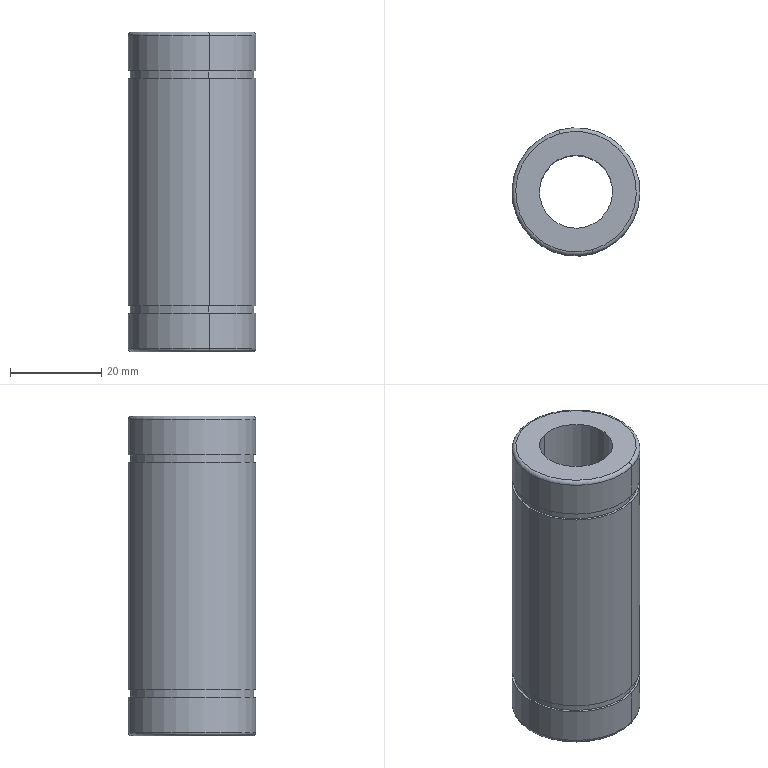Component | SolidWorks | LMUW_N16-3 | 1 solid | 22 faces | box 28 x 28 x 70 mm | volume 28866 mm3 | cylinder 12 | plane 6 | torus 4 | commonest cylinder face diameters 28 x6 27 x4 16 x2
build123d program:
from build123d import *


with BuildPart() as part:
    # Sketch1 → Revolve1 (revolve)
    with BuildSketch(Plane.XY, mode=Mode.PRIVATE) as revolve1_sk:
        with BuildLine():
            Line((0, 13.2), (0, 8))
            Line((0, 8), (70, 8))
            Line((70, 8), (70, 13.2))
            ThreePointArc((70, 13.2), (69.766, 13.766), (69.2, 14))
            Line((69.2, 14), (61.5, 14))
            Line((61.5, 14), (61.5, 13.5))
            Line((61.5, 13.5), (59.9, 13.5))
            Line((59.9, 13.5), (59.9, 14))
            Line((59.9, 14), (10.1, 14))
            Line((10.1, 14), (10.1, 13.5))
            Line((10.1, 13.5), (8.5, 13.5))
            Line((8.5, 13.5), (8.5, 14))
            Line((8.5, 14), (0.8, 14))
            ThreePointArc((0.8, 14), (0.2343, 13.766), (0, 13.2))
        make_face()
    revolve(revolve1_sk.sketch.rotate(Axis((35, 0, 0), (-1, 0, 0)), 270), axis=Axis((35, 0, 0), (-1, 0, 0)))


solid = part.part

# Placed as in the assembly
solid = solid.moved(Location((312, -610.807, 129.441), (0, 90, 0)))
STEP:
#1=COLOUR_RGB('',0.7922,0.8196,0.9333);
#2=FILL_AREA_STYLE_COLOUR('',#1);
#3=FILL_AREA_STYLE('',(#2));
#4=SURFACE_STYLE_FILL_AREA(#3);
#5=SURFACE_SIDE_STYLE('',(#4));
#6=SURFACE_STYLE_USAGE(.BOTH.,#5);
#7=PRESENTATION_STYLE_ASSIGNMENT((#6));
#8=CARTESIAN_POINT('',(12.433,-24.578,4.761));
#9=VERTEX_POINT('',#8);
#10=CARTESIAN_POINT('',(12.134,-23.517,4.761));
#11=VERTEX_POINT('',#10);
#12=CARTESIAN_POINT('',(12.283,-24.048,4.761));
#13=DIRECTION('',(0.,0.,1.));
#14=DIRECTION('',(0.2708,-0.9626,0.));
#15=AXIS2_PLACEMENT_3D('',#12,#13,#14);
#16=CIRCLE('',#15,0.5512);
#17=EDGE_CURVE('',#9,#11,#16,.T.);
#18=ORIENTED_EDGE('',*,*,#17,.T.);
#19=CARTESIAN_POINT('',(12.134,-23.517,5.065));
#20=VERTEX_POINT('',#19);
#21=CARTESIAN_POINT('',(12.134,-23.517,3.718));
#22=DIRECTION('',(0.,0.,1.));
#23=VECTOR('',#22,39.37);
#24=LINE('',#21,#23);
#25=EDGE_CURVE('',#11,#20,#24,.T.);
#26=ORIENTED_EDGE('',*,*,#25,.T.);
#27=CARTESIAN_POINT('',(12.433,-24.578,5.065));
#28=VERTEX_POINT('',#27);
#29=CARTESIAN_POINT('',(12.283,-24.048,5.065));
#30=DIRECTION('',(0.,0.,1.));
#31=DIRECTION('',(0.2708,-0.9626,0.));
#32=AXIS2_PLACEMENT_3D('',#29,#30,#31);
#33=CIRCLE('',#32,0.5512);
#34=EDGE_CURVE('',#28,#20,#33,.T.);
#35=ORIENTED_EDGE('',*,*,#34,.F.);
#36=CARTESIAN_POINT('',(12.433,-24.578,3.718));
#37=DIRECTION('',(0.,0.,1.));
#38=VECTOR('',#37,39.37);
#39=LINE('',#36,#38);
#40=EDGE_CURVE('',#9,#28,#39,.T.);
#41=ORIENTED_EDGE('',*,*,#40,.F.);
#42=EDGE_LOOP('',(#18,#26,#35,#41));
#43=FACE_OUTER_BOUND('',#42,.T.);
#44=CARTESIAN_POINT('',(12.283,-24.048,3.718));
#45=DIRECTION('',(0.,0.,1.));
#46=DIRECTION('',(0.2708,-0.9626,0.));
#47=AXIS2_PLACEMENT_3D('',#44,#45,#46);
#48=CYLINDRICAL_SURFACE('',#47,0.5512);
#49=ADVANCED_FACE('',(#43),#48,.T.);
#50=CARTESIAN_POINT('',(12.427,-24.559,4.698));
#51=VERTEX_POINT('',#50);
#52=CARTESIAN_POINT('',(12.14,-23.536,4.698));
#53=VERTEX_POINT('',#52);
#54=CARTESIAN_POINT('',(12.283,-24.048,4.698));
#55=DIRECTION('',(0.,0.,1.));
#56=DIRECTION('',(0.2708,-0.9626,0.));
#57=AXIS2_PLACEMENT_3D('',#54,#55,#56);
#58=CIRCLE('',#57,0.5315);
#59=EDGE_CURVE('',#51,#53,#58,.T.);
#60=ORIENTED_EDGE('',*,*,#59,.T.);
#61=CARTESIAN_POINT('',(12.14,-23.536,4.761));
#62=VERTEX_POINT('',#61);
#63=CARTESIAN_POINT('',(12.14,-23.536,3.718));
#64=DIRECTION('',(0.,0.,1.));
#65=VECTOR('',#64,39.37);
#66=LINE('',#63,#65);
#67=EDGE_CURVE('',#53,#62,#66,.T.);
#68=ORIENTED_EDGE('',*,*,#67,.T.);
#69=CARTESIAN_POINT('',(12.427,-24.559,4.761));
#70=VERTEX_POINT('',#69);
#71=CARTESIAN_POINT('',(12.283,-24.048,4.761));
#72=DIRECTION('',(0.,0.,1.));
#73=DIRECTION('',(0.2708,-0.9626,0.));
#74=AXIS2_PLACEMENT_3D('',#71,#72,#73);
#75=CIRCLE('',#74,0.5315);
#76=EDGE_CURVE('',#70,#62,#75,.T.);
#77=ORIENTED_EDGE('',*,*,#76,.F.);
#78=CARTESIAN_POINT('',(12.427,-24.559,3.718));
#79=DIRECTION('',(0.,0.,1.));
#80=VECTOR('',#79,39.37);
#81=LINE('',#78,#80);
#82=EDGE_CURVE('',#51,#70,#81,.T.);
#83=ORIENTED_EDGE('',*,*,#82,.F.);
#84=EDGE_LOOP('',(#60,#68,#77,#83));
#85=FACE_OUTER_BOUND('',#84,.T.);
#86=CARTESIAN_POINT('',(12.283,-24.048,3.718));
#87=DIRECTION('',(0.,0.,1.));
#88=DIRECTION('',(0.2708,-0.9626,0.));
#89=AXIS2_PLACEMENT_3D('',#86,#87,#88);
#90=CYLINDRICAL_SURFACE('',#89,0.5315);
#91=ADVANCED_FACE('',(#85),#90,.T.);
#92=CARTESIAN_POINT('',(12.433,-24.578,2.738));
#93=VERTEX_POINT('',#92);
#94=CARTESIAN_POINT('',(12.134,-23.517,2.738));
#95=VERTEX_POINT('',#94);
#96=CARTESIAN_POINT('',(12.283,-24.048,2.738));
#97=DIRECTION('',(0.,0.,1.));
#98=DIRECTION('',(0.2708,-0.9626,0.));
#99=AXIS2_PLACEMENT_3D('',#96,#97,#98);
#100=CIRCLE('',#99,0.5512);
#101=EDGE_CURVE('',#93,#95,#100,.T.);
#102=ORIENTED_EDGE('',*,*,#101,.T.);
#103=CARTESIAN_POINT('',(12.134,-23.517,4.698));
#104=VERTEX_POINT('',#103);
#105=CARTESIAN_POINT('',(12.134,-23.517,3.718));
#106=DIRECTION('',(0.,0.,1.));
#107=VECTOR('',#106,39.37);
#108=LINE('',#105,#107);
#109=EDGE_CURVE('',#95,#104,#108,.T.);
#110=ORIENTED_EDGE('',*,*,#109,.T.);
#111=CARTESIAN_POINT('',(12.433,-24.578,4.698));
#112=VERTEX_POINT('',#111);
#113=CARTESIAN_POINT('',(12.283,-24.048,4.698));
#114=DIRECTION('',(0.,0.,1.));
#115=DIRECTION('',(0.2708,-0.9626,0.));
#116=AXIS2_PLACEMENT_3D('',#113,#114,#115);
#117=CIRCLE('',#116,0.5512);
#118=EDGE_CURVE('',#112,#104,#117,.T.);
#119=ORIENTED_EDGE('',*,*,#118,.F.);
#120=CARTESIAN_POINT('',(12.433,-24.578,3.718));
#121=DIRECTION('',(0.,0.,1.));
#122=VECTOR('',#121,39.37);
#123=LINE('',#120,#122);
#124=EDGE_CURVE('',#93,#112,#123,.T.);
#125=ORIENTED_EDGE('',*,*,#124,.F.);
#126=EDGE_LOOP('',(#102,#110,#119,#125));
#127=FACE_OUTER_BOUND('',#126,.T.);
#128=CARTESIAN_POINT('',(12.283,-24.048,3.718));
#129=DIRECTION('',(0.,0.,1.));
#130=DIRECTION('',(0.2708,-0.9626,0.));
#131=AXIS2_PLACEMENT_3D('',#128,#129,#130);
#132=CYLINDRICAL_SURFACE('',#131,0.5512);
#133=ADVANCED_FACE('',(#127),#132,.T.);
#134=CARTESIAN_POINT('',(12.427,-24.559,2.675));
#135=VERTEX_POINT('',#134);
#136=CARTESIAN_POINT('',(12.14,-23.536,2.675));
#137=VERTEX_POINT('',#136);
#138=CARTESIAN_POINT('',(12.283,-24.048,2.675));
#139=DIRECTION('',(0.,0.,1.));
#140=DIRECTION('',(0.2708,-0.9626,0.));
#141=AXIS2_PLACEMENT_3D('',#138,#139,#140);
#142=CIRCLE('',#141,0.5315);
#143=EDGE_CURVE('',#135,#137,#142,.T.);
#144=ORIENTED_EDGE('',*,*,#143,.T.);
#145=CARTESIAN_POINT('',(12.14,-23.536,2.738));
#146=VERTEX_POINT('',#145);
#147=CARTESIAN_POINT('',(12.14,-23.536,3.718));
#148=DIRECTION('',(0.,0.,1.));
#149=VECTOR('',#148,39.37);
#150=LINE('',#147,#149);
#151=EDGE_CURVE('',#137,#146,#150,.T.);
#152=ORIENTED_EDGE('',*,*,#151,.T.);
#153=CARTESIAN_POINT('',(12.427,-24.559,2.738));
#154=VERTEX_POINT('',#153);
#155=CARTESIAN_POINT('',(12.283,-24.048,2.738));
#156=DIRECTION('',(0.,0.,1.));
#157=DIRECTION('',(0.2708,-0.9626,0.));
#158=AXIS2_PLACEMENT_3D('',#155,#156,#157);
#159=CIRCLE('',#158,0.5315);
#160=EDGE_CURVE('',#154,#146,#159,.T.);
#161=ORIENTED_EDGE('',*,*,#160,.F.);
#162=CARTESIAN_POINT('',(12.427,-24.559,3.718));
#163=DIRECTION('',(0.,0.,1.));
#164=VECTOR('',#163,39.37);
#165=LINE('',#162,#164);
#166=EDGE_CURVE('',#135,#154,#165,.T.);
#167=ORIENTED_EDGE('',*,*,#166,.F.);
#168=EDGE_LOOP('',(#144,#152,#161,#167));
#169=FACE_OUTER_BOUND('',#168,.T.);
#170=CARTESIAN_POINT('',(12.283,-24.048,3.718));
#171=DIRECTION('',(0.,0.,1.));
#172=DIRECTION('',(0.2708,-0.9626,0.));
#173=AXIS2_PLACEMENT_3D('',#170,#171,#172);
#174=CYLINDRICAL_SURFACE('',#173,0.5315);
#175=ADVANCED_FACE('',(#169),#174,.T.);
#176=CARTESIAN_POINT('',(12.433,-24.578,2.372));
#177=VERTEX_POINT('',#176);
#178=CARTESIAN_POINT('',(12.134,-23.517,2.372));
#179=VERTEX_POINT('',#178);
#180=CARTESIAN_POINT('',(12.283,-24.048,2.372));
#181=DIRECTION('',(0.,0.,1.));
#182=DIRECTION('',(0.2708,-0.9626,0.));
#183=AXIS2_PLACEMENT_3D('',#180,#181,#182);
#184=CIRCLE('',#183,0.5512);
#185=EDGE_CURVE('',#177,#179,#184,.T.);
#186=ORIENTED_EDGE('',*,*,#185,.T.);
#187=CARTESIAN_POINT('',(12.134,-23.517,2.675));
#188=VERTEX_POINT('',#187);
#189=CARTESIAN_POINT('',(12.134,-23.517,3.718));
#190=DIRECTION('',(0.,0.,1.));
#191=VECTOR('',#190,39.37);
#192=LINE('',#189,#191);
#193=EDGE_CURVE('',#179,#188,#192,.T.);
#194=ORIENTED_EDGE('',*,*,#193,.T.);
#195=CARTESIAN_POINT('',(12.433,-24.578,2.675));
#196=VERTEX_POINT('',#195);
#197=CARTESIAN_POINT('',(12.283,-24.048,2.675));
#198=DIRECTION('',(0.,0.,1.));
#199=DIRECTION('',(0.2708,-0.9626,0.));
#200=AXIS2_PLACEMENT_3D('',#197,#198,#199);
#201=CIRCLE('',#200,0.5512);
#202=EDGE_CURVE('',#196,#188,#201,.T.);
#203=ORIENTED_EDGE('',*,*,#202,.F.);
#204=CARTESIAN_POINT('',(12.433,-24.578,3.718));
#205=DIRECTION('',(0.,0.,1.));
#206=VECTOR('',#205,39.37);
#207=LINE('',#204,#206);
#208=EDGE_CURVE('',#177,#196,#207,.T.);
#209=ORIENTED_EDGE('',*,*,#208,.F.);
#210=EDGE_LOOP('',(#186,#194,#203,#209));
#211=FACE_OUTER_BOUND('',#210,.T.);
#212=CARTESIAN_POINT('',(12.283,-24.048,3.718));
#213=DIRECTION('',(0.,0.,1.));
#214=DIRECTION('',(0.2708,-0.9626,0.));
#215=AXIS2_PLACEMENT_3D('',#212,#213,#214);
#216=CYLINDRICAL_SURFACE('',#215,0.5512);
#217=ADVANCED_FACE('',(#211),#216,.T.);
#218=CARTESIAN_POINT('',(12.424,-24.548,2.34));
#219=VERTEX_POINT('',#218);
#220=CARTESIAN_POINT('',(12.143,-23.547,2.34));
#221=VERTEX_POINT('',#220);
#222=CARTESIAN_POINT('',(12.283,-24.048,2.34));
#223=DIRECTION('',(0.,0.,1.));
#224=DIRECTION('',(0.2708,-0.9626,0.));
#225=AXIS2_PLACEMENT_3D('',#222,#223,#224);
#226=CIRCLE('',#225,0.5197);
#227=EDGE_CURVE('',#219,#221,#226,.T.);
#228=ORIENTED_EDGE('',*,*,#227,.T.);
#229=CARTESIAN_POINT('',(12.143,-23.547,2.372));
#230=DIRECTION('',(0.9626,0.2708,-0.));
#231=DIRECTION('',(-0.2708,0.9626,0.));
#232=AXIS2_PLACEMENT_3D('',#229,#230,#231);
#233=CIRCLE('',#232,0.0315);
#234=EDGE_CURVE('',#221,#179,#233,.T.);
#235=ORIENTED_EDGE('',*,*,#234,.T.);
#236=ORIENTED_EDGE('',*,*,#185,.F.);
#237=CARTESIAN_POINT('',(12.424,-24.548,2.372));
#238=DIRECTION('',(-0.9626,-0.2708,0.));
#239=DIRECTION('',(0.2708,-0.9626,0.));
#240=AXIS2_PLACEMENT_3D('',#237,#238,#239);
#241=CIRCLE('',#240,0.0315);
#242=EDGE_CURVE('',#219,#177,#241,.T.);
#243=ORIENTED_EDGE('',*,*,#242,.F.);
#244=EDGE_LOOP('',(#228,#235,#236,#243));
#245=FACE_OUTER_BOUND('',#244,.T.);
#246=CARTESIAN_POINT('',(12.283,-24.048,2.372));
#247=DIRECTION('',(0.,0.,1.));
#248=DIRECTION('',(0.2708,-0.9626,0.));
#249=AXIS2_PLACEMENT_3D('',#246,#247,#248);
#250=TOROIDAL_SURFACE('',#249,0.5197,0.0315);
#251=ADVANCED_FACE('',(#245),#250,.T.);
#252=CARTESIAN_POINT('',(12.198,-23.744,2.34));
#253=VERTEX_POINT('',#252);
#254=CARTESIAN_POINT('',(12.369,-24.351,2.34));
#255=VERTEX_POINT('',#254);
#256=CARTESIAN_POINT('',(12.283,-24.048,2.34));
#257=DIRECTION('',(0.,0.,1.));
#258=DIRECTION('',(0.2708,-0.9626,0.));
#259=AXIS2_PLACEMENT_3D('',#256,#257,#258);
#260=CIRCLE('',#259,0.315);
#261=EDGE_CURVE('',#253,#255,#260,.T.);
#262=ORIENTED_EDGE('',*,*,#261,.F.);
#263=CARTESIAN_POINT('',(12.198,-23.744,5.096));
#264=VERTEX_POINT('',#263);
#265=CARTESIAN_POINT('',(12.198,-23.744,3.718));
#266=DIRECTION('',(0.,0.,1.));
#267=VECTOR('',#266,39.37);
#268=LINE('',#265,#267);
#269=EDGE_CURVE('',#253,#264,#268,.T.);
#270=ORIENTED_EDGE('',*,*,#269,.T.);
#271=CARTESIAN_POINT('',(12.369,-24.351,5.096));
#272=VERTEX_POINT('',#271);
#273=CARTESIAN_POINT('',(12.283,-24.048,5.096));
#274=DIRECTION('',(0.,0.,1.));
#275=DIRECTION('',(0.2708,-0.9626,0.));
#276=AXIS2_PLACEMENT_3D('',#273,#274,#275);
#277=CIRCLE('',#276,0.315);
#278=EDGE_CURVE('',#264,#272,#277,.T.);
#279=ORIENTED_EDGE('',*,*,#278,.T.);
#280=CARTESIAN_POINT('',(12.369,-24.351,3.718));
#281=DIRECTION('',(0.,0.,1.));
#282=VECTOR('',#281,39.37);
#283=LINE('',#280,#282);
#284=EDGE_CURVE('',#255,#272,#283,.T.);
#285=ORIENTED_EDGE('',*,*,#284,.F.);
#286=EDGE_LOOP('',(#262,#270,#279,#285));
#287=FACE_OUTER_BOUND('',#286,.T.);
#288=CARTESIAN_POINT('',(12.283,-24.048,3.718));
#289=DIRECTION('',(0.,0.,1.));
#290=DIRECTION('',(0.2708,-0.9626,0.));
#291=AXIS2_PLACEMENT_3D('',#288,#289,#290);
#292=CYLINDRICAL_SURFACE('',#291,0.315);
#293=ADVANCED_FACE('',(#287),#292,.F.);
#294=ORIENTED_EDGE('',*,*,#34,.T.);
#295=CARTESIAN_POINT('',(12.143,-23.547,5.096));
#296=VERTEX_POINT('',#295);
#297=CARTESIAN_POINT('',(12.143,-23.547,5.065));
#298=DIRECTION('',(0.9626,0.2708,-0.));
#299=DIRECTION('',(-0.2708,0.9626,0.));
#300=AXIS2_PLACEMENT_3D('',#297,#298,#299);
#301=CIRCLE('',#300,0.0315);
#302=EDGE_CURVE('',#20,#296,#301,.T.);
#303=ORIENTED_EDGE('',*,*,#302,.T.);
#304=CARTESIAN_POINT('',(12.424,-24.548,5.096));
#305=VERTEX_POINT('',#304);
#306=CARTESIAN_POINT('',(12.283,-24.048,5.096));
#307=DIRECTION('',(0.,0.,1.));
#308=DIRECTION('',(0.2708,-0.9626,0.));
#309=AXIS2_PLACEMENT_3D('',#306,#307,#308);
#310=CIRCLE('',#309,0.5197);
#311=EDGE_CURVE('',#305,#296,#310,.T.);
#312=ORIENTED_EDGE('',*,*,#311,.F.);
#313=CARTESIAN_POINT('',(12.424,-24.548,5.065));
#314=DIRECTION('',(-0.9626,-0.2708,0.));
#315=DIRECTION('',(0.2708,-0.9626,0.));
#316=AXIS2_PLACEMENT_3D('',#313,#314,#315);
#317=CIRCLE('',#316,0.0315);
#318=EDGE_CURVE('',#28,#305,#317,.T.);
#319=ORIENTED_EDGE('',*,*,#318,.F.);
#320=EDGE_LOOP('',(#294,#303,#312,#319));
#321=FACE_OUTER_BOUND('',#320,.T.);
#322=CARTESIAN_POINT('',(12.283,-24.048,5.065));
#323=DIRECTION('',(0.,0.,1.));
#324=DIRECTION('',(0.2708,-0.9626,0.));
#325=AXIS2_PLACEMENT_3D('',#322,#323,#324);
#326=TOROIDAL_SURFACE('',#325,0.5197,0.0315);
#327=ADVANCED_FACE('',(#321),#326,.T.);
#328=ORIENTED_EDGE('',*,*,#302,.F.);
#329=CARTESIAN_POINT('',(12.283,-24.048,5.065));
#330=DIRECTION('',(0.,0.,1.));
#331=DIRECTION('',(0.2708,-0.9626,0.));
#332=AXIS2_PLACEMENT_3D('',#329,#330,#331);
#333=CIRCLE('',#332,0.5512);
#334=EDGE_CURVE('',#20,#28,#333,.T.);
#335=ORIENTED_EDGE('',*,*,#334,.T.);
#336=ORIENTED_EDGE('',*,*,#318,.T.);
#337=CARTESIAN_POINT('',(12.283,-24.048,5.096));
#338=DIRECTION('',(0.,0.,1.));
#339=DIRECTION('',(0.2708,-0.9626,0.));
#340=AXIS2_PLACEMENT_3D('',#337,#338,#339);
#341=CIRCLE('',#340,0.5197);
#342=EDGE_CURVE('',#296,#305,#341,.T.);
#343=ORIENTED_EDGE('',*,*,#342,.F.);
#344=EDGE_LOOP('',(#328,#335,#336,#343));
#345=FACE_OUTER_BOUND('',#344,.T.);
#346=CARTESIAN_POINT('',(12.283,-24.048,5.065));
#347=DIRECTION('',(0.,0.,1.));
#348=DIRECTION('',(0.2708,-0.9626,0.));
#349=AXIS2_PLACEMENT_3D('',#346,#347,#348);
#350=TOROIDAL_SURFACE('',#349,0.5197,0.0315);
#351=ADVANCED_FACE('',(#345),#350,.T.);
#352=CARTESIAN_POINT('',(12.283,-24.048,5.096));
#353=DIRECTION('',(0.,0.,1.));
#354=DIRECTION('',(0.2708,-0.9626,0.));
#355=AXIS2_PLACEMENT_3D('',#352,#353,#354);
#356=CIRCLE('',#355,0.315);
#357=EDGE_CURVE('',#272,#264,#356,.T.);
#358=ORIENTED_EDGE('',*,*,#357,.F.);
#359=ORIENTED_EDGE('',*,*,#278,.F.);
#360=EDGE_LOOP('',(#358,#359));
#361=FACE_BOUND('',#360,.T.);
#362=ORIENTED_EDGE('',*,*,#311,.T.);
#363=ORIENTED_EDGE('',*,*,#342,.T.);
#364=EDGE_LOOP('',(#362,#363));
#365=FACE_OUTER_BOUND('',#364,.T.);
#366=CARTESIAN_POINT('',(12.784,-23.907,5.096));
#367=DIRECTION('',(-0.,-0.,-1.));
#368=DIRECTION('',(-0.2708,0.9626,-0.));
#369=AXIS2_PLACEMENT_3D('',#366,#367,#368);
#370=PLANE('',#369);
#371=ADVANCED_FACE('',(#361,#365),#370,.F.);
#372=ORIENTED_EDGE('',*,*,#269,.F.);
#373=CARTESIAN_POINT('',(12.283,-24.048,2.34));
#374=DIRECTION('',(0.,0.,1.));
#375=DIRECTION('',(0.2708,-0.9626,0.));
#376=AXIS2_PLACEMENT_3D('',#373,#374,#375);
#377=CIRCLE('',#376,0.315);
#378=EDGE_CURVE('',#255,#253,#377,.T.);
#379=ORIENTED_EDGE('',*,*,#378,.F.);
#380=ORIENTED_EDGE('',*,*,#284,.T.);
#381=ORIENTED_EDGE('',*,*,#357,.T.);
#382=EDGE_LOOP('',(#372,#379,#380,#381));
#383=FACE_OUTER_BOUND('',#382,.T.);
#384=CARTESIAN_POINT('',(12.283,-24.048,3.718));
#385=DIRECTION('',(0.,0.,1.));
#386=DIRECTION('',(0.2708,-0.9626,0.));
#387=AXIS2_PLACEMENT_3D('',#384,#385,#386);
#388=CYLINDRICAL_SURFACE('',#387,0.315);
#389=ADVANCED_FACE('',(#383),#388,.F.);
#390=ORIENTED_EDGE('',*,*,#227,.F.);
#391=CARTESIAN_POINT('',(12.283,-24.048,2.34));
#392=DIRECTION('',(0.,0.,1.));
#393=DIRECTION('',(0.2708,-0.9626,0.));
#394=AXIS2_PLACEMENT_3D('',#391,#392,#393);
#395=CIRCLE('',#394,0.5197);
#396=EDGE_CURVE('',#221,#219,#395,.T.);
#397=ORIENTED_EDGE('',*,*,#396,.F.);
#398=EDGE_LOOP('',(#390,#397));
#399=FACE_OUTER_BOUND('',#398,.T.);
#400=ORIENTED_EDGE('',*,*,#378,.T.);
#401=ORIENTED_EDGE('',*,*,#261,.T.);
#402=EDGE_LOOP('',(#400,#401));
#403=FACE_BOUND('',#402,.T.);
#404=CARTESIAN_POINT('',(12.587,-23.962,2.34));
#405=DIRECTION('',(0.,0.,1.));
#406=DIRECTION('',(0.2708,-0.9626,0.));
#407=AXIS2_PLACEMENT_3D('',#404,#405,#406);
#408=PLANE('',#407);
#409=ADVANCED_FACE('',(#399,#403),#408,.F.);
#410=ORIENTED_EDGE('',*,*,#234,.F.);
#411=ORIENTED_EDGE('',*,*,#396,.T.);
#412=ORIENTED_EDGE('',*,*,#242,.T.);
#413=CARTESIAN_POINT('',(12.283,-24.048,2.372));
#414=DIRECTION('',(0.,0.,1.));
#415=DIRECTION('',(0.2708,-0.9626,0.));
#416=AXIS2_PLACEMENT_3D('',#413,#414,#415);
#417=CIRCLE('',#416,0.5512);
#418=EDGE_CURVE('',#179,#177,#417,.T.);
#419=ORIENTED_EDGE('',*,*,#418,.F.);
#420=EDGE_LOOP('',(#410,#411,#412,#419));
#421=FACE_OUTER_BOUND('',#420,.T.);
#422=CARTESIAN_POINT('',(12.283,-24.048,2.372));
#423=DIRECTION('',(0.,0.,1.));
#424=DIRECTION('',(0.2708,-0.9626,0.));
#425=AXIS2_PLACEMENT_3D('',#422,#423,#424);
#426=TOROIDAL_SURFACE('',#425,0.5197,0.0315);
#427=ADVANCED_FACE('',(#421),#426,.T.);
#428=ORIENTED_EDGE('',*,*,#193,.F.);
#429=ORIENTED_EDGE('',*,*,#418,.T.);
#430=ORIENTED_EDGE('',*,*,#208,.T.);
#431=CARTESIAN_POINT('',(12.283,-24.048,2.675));
#432=DIRECTION('',(0.,0.,1.));
#433=DIRECTION('',(0.2708,-0.9626,0.));
#434=AXIS2_PLACEMENT_3D('',#431,#432,#433);
#435=CIRCLE('',#434,0.5512);
#436=EDGE_CURVE('',#188,#196,#435,.T.);
#437=ORIENTED_EDGE('',*,*,#436,.F.);
#438=EDGE_LOOP('',(#428,#429,#430,#437));
#439=FACE_OUTER_BOUND('',#438,.T.);
#440=CARTESIAN_POINT('',(12.283,-24.048,3.718));
#441=DIRECTION('',(0.,0.,1.));
#442=DIRECTION('',(0.2708,-0.9626,0.));
#443=AXIS2_PLACEMENT_3D('',#440,#441,#442);
#444=CYLINDRICAL_SURFACE('',#443,0.5512);
#445=ADVANCED_FACE('',(#439),#444,.T.);
#446=ORIENTED_EDGE('',*,*,#143,.F.);
#447=CARTESIAN_POINT('',(12.283,-24.048,2.675));
#448=DIRECTION('',(0.,0.,1.));
#449=DIRECTION('',(0.2708,-0.9626,0.));
#450=AXIS2_PLACEMENT_3D('',#447,#448,#449);
#451=CIRCLE('',#450,0.5315);
#452=EDGE_CURVE('',#137,#135,#451,.T.);
#453=ORIENTED_EDGE('',*,*,#452,.F.);
#454=EDGE_LOOP('',(#446,#453));
#455=FACE_BOUND('',#454,.T.);
#456=ORIENTED_EDGE('',*,*,#202,.T.);
#457=ORIENTED_EDGE('',*,*,#436,.T.);
#458=EDGE_LOOP('',(#456,#457));
#459=FACE_OUTER_BOUND('',#458,.T.);
#460=CARTESIAN_POINT('',(12.814,-23.898,2.675));
#461=DIRECTION('',(-0.,-0.,-1.));
#462=DIRECTION('',(-0.2708,0.9626,-0.));
#463=AXIS2_PLACEMENT_3D('',#460,#461,#462);
#464=PLANE('',#463);
#465=ADVANCED_FACE('',(#455,#459),#464,.F.);
#466=ORIENTED_EDGE('',*,*,#151,.F.);
#467=ORIENTED_EDGE('',*,*,#452,.T.);
#468=ORIENTED_EDGE('',*,*,#166,.T.);
#469=CARTESIAN_POINT('',(12.283,-24.048,2.738));
#470=DIRECTION('',(0.,0.,1.));
#471=DIRECTION('',(0.2708,-0.9626,0.));
#472=AXIS2_PLACEMENT_3D('',#469,#470,#471);
#473=CIRCLE('',#472,0.5315);
#474=EDGE_CURVE('',#146,#154,#473,.T.);
#475=ORIENTED_EDGE('',*,*,#474,.F.);
#476=EDGE_LOOP('',(#466,#467,#468,#475));
#477=FACE_OUTER_BOUND('',#476,.T.);
#478=CARTESIAN_POINT('',(12.283,-24.048,3.718));
#479=DIRECTION('',(0.,0.,1.));
#480=DIRECTION('',(0.2708,-0.9626,0.));
#481=AXIS2_PLACEMENT_3D('',#478,#479,#480);
#482=CYLINDRICAL_SURFACE('',#481,0.5315);
#483=ADVANCED_FACE('',(#477),#482,.T.);
#484=ORIENTED_EDGE('',*,*,#101,.F.);
#485=CARTESIAN_POINT('',(12.283,-24.048,2.738));
#486=DIRECTION('',(0.,0.,1.));
#487=DIRECTION('',(0.2708,-0.9626,0.));
#488=AXIS2_PLACEMENT_3D('',#485,#486,#487);
#489=CIRCLE('',#488,0.5512);
#490=EDGE_CURVE('',#95,#93,#489,.T.);
#491=ORIENTED_EDGE('',*,*,#490,.F.);
#492=EDGE_LOOP('',(#484,#491));
#493=FACE_OUTER_BOUND('',#492,.T.);
#494=ORIENTED_EDGE('',*,*,#160,.T.);
#495=ORIENTED_EDGE('',*,*,#474,.T.);
#496=EDGE_LOOP('',(#494,#495));
#497=FACE_BOUND('',#496,.T.);
#498=CARTESIAN_POINT('',(12.795,-23.904,2.738));
#499=DIRECTION('',(0.,0.,1.));
#500=DIRECTION('',(0.2708,-0.9626,0.));
#501=AXIS2_PLACEMENT_3D('',#498,#499,#500);
#502=PLANE('',#501);
#503=ADVANCED_FACE('',(#493,#497),#502,.F.);
#504=ORIENTED_EDGE('',*,*,#109,.F.);
#505=ORIENTED_EDGE('',*,*,#490,.T.);
#506=ORIENTED_EDGE('',*,*,#124,.T.);
#507=CARTESIAN_POINT('',(12.283,-24.048,4.698));
#508=DIRECTION('',(0.,0.,1.));
#509=DIRECTION('',(0.2708,-0.9626,0.));
#510=AXIS2_PLACEMENT_3D('',#507,#508,#509);
#511=CIRCLE('',#510,0.5512);
#512=EDGE_CURVE('',#104,#112,#511,.T.);
#513=ORIENTED_EDGE('',*,*,#512,.F.);
#514=EDGE_LOOP('',(#504,#505,#506,#513));
#515=FACE_OUTER_BOUND('',#514,.T.);
#516=CARTESIAN_POINT('',(12.283,-24.048,3.718));
#517=DIRECTION('',(0.,0.,1.));
#518=DIRECTION('',(0.2708,-0.9626,0.));
#519=AXIS2_PLACEMENT_3D('',#516,#517,#518);
#520=CYLINDRICAL_SURFACE('',#519,0.5512);
#521=ADVANCED_FACE('',(#515),#520,.T.);
#522=ORIENTED_EDGE('',*,*,#59,.F.);
#523=CARTESIAN_POINT('',(12.283,-24.048,4.698));
#524=DIRECTION('',(0.,0.,1.));
#525=DIRECTION('',(0.2708,-0.9626,0.));
#526=AXIS2_PLACEMENT_3D('',#523,#524,#525);
#527=CIRCLE('',#526,0.5315);
#528=EDGE_CURVE('',#53,#51,#527,.T.);
#529=ORIENTED_EDGE('',*,*,#528,.F.);
#530=EDGE_LOOP('',(#522,#529));
#531=FACE_BOUND('',#530,.T.);
#532=ORIENTED_EDGE('',*,*,#118,.T.);
#533=ORIENTED_EDGE('',*,*,#512,.T.);
#534=EDGE_LOOP('',(#532,#533));
#535=FACE_OUTER_BOUND('',#534,.T.);
#536=CARTESIAN_POINT('',(12.814,-23.898,4.698));
#537=DIRECTION('',(-0.,-0.,-1.));
#538=DIRECTION('',(-0.2708,0.9626,-0.));
#539=AXIS2_PLACEMENT_3D('',#536,#537,#538);
#540=PLANE('',#539);
#541=ADVANCED_FACE('',(#531,#535),#540,.F.);
#542=ORIENTED_EDGE('',*,*,#67,.F.);
#543=ORIENTED_EDGE('',*,*,#528,.T.);
#544=ORIENTED_EDGE('',*,*,#82,.T.);
#545=CARTESIAN_POINT('',(12.283,-24.048,4.761));
#546=DIRECTION('',(0.,0.,1.));
#547=DIRECTION('',(0.2708,-0.9626,0.));
#548=AXIS2_PLACEMENT_3D('',#545,#546,#547);
#549=CIRCLE('',#548,0.5315);
#550=EDGE_CURVE('',#62,#70,#549,.T.);
#551=ORIENTED_EDGE('',*,*,#550,.F.);
#552=EDGE_LOOP('',(#542,#543,#544,#551));
#553=FACE_OUTER_BOUND('',#552,.T.);
#554=CARTESIAN_POINT('',(12.283,-24.048,3.718));
#555=DIRECTION('',(0.,0.,1.));
#556=DIRECTION('',(0.2708,-0.9626,0.));
#557=AXIS2_PLACEMENT_3D('',#554,#555,#556);
#558=CYLINDRICAL_SURFACE('',#557,0.5315);
#559=ADVANCED_FACE('',(#553),#558,.T.);
#560=ORIENTED_EDGE('',*,*,#17,.F.);
#561=CARTESIAN_POINT('',(12.283,-24.048,4.761));
#562=DIRECTION('',(0.,0.,1.));
#563=DIRECTION('',(0.2708,-0.9626,0.));
#564=AXIS2_PLACEMENT_3D('',#561,#562,#563);
#565=CIRCLE('',#564,0.5512);
#566=EDGE_CURVE('',#11,#9,#565,.T.);
#567=ORIENTED_EDGE('',*,*,#566,.F.);
#568=EDGE_LOOP('',(#560,#567));
#569=FACE_OUTER_BOUND('',#568,.T.);
#570=ORIENTED_EDGE('',*,*,#76,.T.);
#571=ORIENTED_EDGE('',*,*,#550,.T.);
#572=EDGE_LOOP('',(#570,#571));
#573=FACE_BOUND('',#572,.T.);
#574=CARTESIAN_POINT('',(12.795,-23.904,4.761));
#575=DIRECTION('',(0.,0.,1.));
#576=DIRECTION('',(0.2708,-0.9626,0.));
#577=AXIS2_PLACEMENT_3D('',#574,#575,#576);
#578=PLANE('',#577);
#579=ADVANCED_FACE('',(#569,#573),#578,.F.);
#580=ORIENTED_EDGE('',*,*,#25,.F.);
#581=ORIENTED_EDGE('',*,*,#566,.T.);
#582=ORIENTED_EDGE('',*,*,#40,.T.);
#583=ORIENTED_EDGE('',*,*,#334,.F.);
#584=EDGE_LOOP('',(#580,#581,#582,#583));
#585=FACE_OUTER_BOUND('',#584,.T.);
#586=CARTESIAN_POINT('',(12.283,-24.048,3.718));
#587=DIRECTION('',(0.,0.,1.));
#588=DIRECTION('',(0.2708,-0.9626,0.));
#589=AXIS2_PLACEMENT_3D('',#586,#587,#588);
#590=CYLINDRICAL_SURFACE('',#589,0.5512);
#591=ADVANCED_FACE('',(#585),#590,.T.);
#592=CLOSED_SHELL('',(#49,#91,#133,#175,#217,#251,#293,#327,#351,#371,#389,#409,#427,#445,#465,#483,#503,#521,#541,#559,#579,#591));
#593=MANIFOLD_SOLID_BREP('',#592);
#594=STYLED_ITEM('',(#7),#593);
#595=(LENGTH_UNIT()NAMED_UNIT(*)SI_UNIT($,.METRE.));
#596=LENGTH_MEASURE_WITH_UNIT(LENGTH_MEASURE(0.0254),#595);
#597=DIMENSIONAL_EXPONENTS(1.,0.,0.,0.,0.,0.,0.);
#598=(CONVERSION_BASED_UNIT('',#596)LENGTH_UNIT()NAMED_UNIT(#597));
#599=UNCERTAINTY_MEASURE_WITH_UNIT(LENGTH_MEASURE(0.00001),#598,'','');
#600=(NAMED_UNIT(*)PLANE_ANGLE_UNIT()SI_UNIT($,.RADIAN.));
#601=(NAMED_UNIT(*)SI_UNIT($,.STERADIAN.)SOLID_ANGLE_UNIT());
#602=(GEOMETRIC_REPRESENTATION_CONTEXT(3)GLOBAL_UNCERTAINTY_ASSIGNED_CONTEXT((#599))GLOBAL_UNIT_ASSIGNED_CONTEXT((#598,#600,#601))REPRESENTATION_CONTEXT('',''));
#603=MECHANICAL_DESIGN_GEOMETRIC_PRESENTATION_REPRESENTATION('',(#594),#602);
#604=PRESENTATION_LAYER_ASSIGNMENT('','',(#594));
#605=CARTESIAN_POINT('',(0.,0.,0.));
#606=DIRECTION('',(0.,0.,1.));
#607=DIRECTION('',(1.,0.,0.));
#608=AXIS2_PLACEMENT_3D('',#605,#606,#607);
#609=(LENGTH_UNIT()NAMED_UNIT(*)SI_UNIT($,.METRE.));
#610=LENGTH_MEASURE_WITH_UNIT(LENGTH_MEASURE(0.0254),#609);
#611=DIMENSIONAL_EXPONENTS(1.,0.,0.,0.,0.,0.,0.);
#612=(CONVERSION_BASED_UNIT('',#610)LENGTH_UNIT()NAMED_UNIT(#611));
#613=UNCERTAINTY_MEASURE_WITH_UNIT(LENGTH_MEASURE(0.00001),#612,'','');
#614=(NAMED_UNIT(*)PLANE_ANGLE_UNIT()SI_UNIT($,.RADIAN.));
#615=(NAMED_UNIT(*)SI_UNIT($,.STERADIAN.)SOLID_ANGLE_UNIT());
#616=(GEOMETRIC_REPRESENTATION_CONTEXT(3)GLOBAL_UNCERTAINTY_ASSIGNED_CONTEXT((#613))GLOBAL_UNIT_ASSIGNED_CONTEXT((#612,#614,#615))REPRESENTATION_CONTEXT('',''));
#617=ADVANCED_BREP_SHAPE_REPRESENTATION('',(#593,#608),#616);